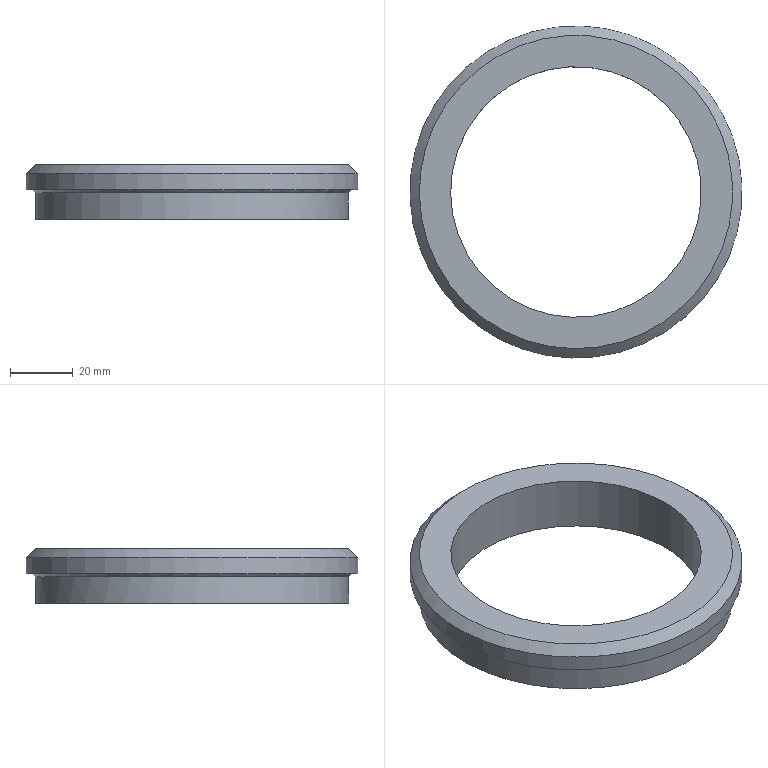Component | NX | CA6140-ZHUZHOU-ZHOUTAO2 | 1 solid | 8 faces | box 106 x 106 x 17.5 mm | volume 55934 mm3 | plane 3 | cylinder 3 | cone 2 | commonest cylinder face diameters 100 x1 80 x1 106 x1
STEP:
#1=CARTESIAN_POINT('',(0.,0.,0.));
#2=DIRECTION('',(0.,0.,1.));
#3=DIRECTION('',(1.,0.,0.));
#4=AXIS2_PLACEMENT_3D('',#1,#2,#3);
#5=CARTESIAN_POINT('',(-29.389,-40.451,-315.951));
#6=VERTEX_POINT('',#5);
#7=CARTESIAN_POINT('',(0.,-0.,-315.951));
#8=DIRECTION('',(0.,0.,1.));
#9=DIRECTION('',(-0.5878,-0.809,0.));
#10=AXIS2_PLACEMENT_3D('',#7,#8,#9);
#11=CIRCLE('',#10,50.);
#12=CARTESIAN_POINT('',(0.,-0.,-315.951));
#13=DIRECTION('',(0.,0.,1.));
#14=DIRECTION('',(-0.5878,-0.809,0.));
#15=AXIS2_PLACEMENT_3D('',#12,#13,#14);
#16=PLANE('',#15);
#17=CARTESIAN_POINT('',(0.,0.));
#18=DIRECTION('',(1.,0.));
#19=AXIS2_PLACEMENT_2D('',#17,#18);
#20=CIRCLE('',#19,50.);
#21=(GEOMETRIC_REPRESENTATION_CONTEXT(2)PARAMETRIC_REPRESENTATION_CONTEXT()REPRESENTATION_CONTEXT('',''));
#22=DEFINITIONAL_REPRESENTATION('',(#20),#21);
#23=PCURVE('',#16,#22);
#24=CARTESIAN_POINT('',(0.,-0.,-318.951));
#25=DIRECTION('',(0.,0.,-1.));
#26=DIRECTION('',(0.5878,0.809,0.));
#27=AXIS2_PLACEMENT_3D('',#24,#25,#26);
#28=CONICAL_SURFACE('',#27,53.,0.7854);
#29=CARTESIAN_POINT('',(9.425,-3.));
#30=DIRECTION('',(-1.,0.));
#31=VECTOR('',#30,1.);
#32=LINE('',#29,#31);
#33=(GEOMETRIC_REPRESENTATION_CONTEXT(2)PARAMETRIC_REPRESENTATION_CONTEXT()REPRESENTATION_CONTEXT('',''));
#34=DEFINITIONAL_REPRESENTATION('',(#32),#33);
#35=PCURVE('',#28,#34);
#36=SURFACE_CURVE('',#11,(#23,#35),.PCURVE_S1.);
#37=EDGE_CURVE('',#6,#6,#36,.T.);
#38=ORIENTED_EDGE('',*,*,#37,.T.);
#39=EDGE_LOOP('',(#38));
#40=FACE_BOUND('',#39,.T.);
#41=CARTESIAN_POINT('',(23.511,32.361,-315.951));
#42=VERTEX_POINT('',#41);
#43=CARTESIAN_POINT('',(0.,-0.,-315.951));
#44=DIRECTION('',(0.,0.,-1.));
#45=DIRECTION('',(0.5878,0.809,0.));
#46=AXIS2_PLACEMENT_3D('',#43,#44,#45);
#47=CIRCLE('',#46,40.);
#48=CARTESIAN_POINT('',(-40.,0.));
#49=CARTESIAN_POINT('',(-40.,69.282));
#50=CARTESIAN_POINT('',(20.,34.641));
#51=CARTESIAN_POINT('',(80.,0.));
#52=CARTESIAN_POINT('',(20.,-34.641));
#53=CARTESIAN_POINT('',(-40.,-69.282));
#54=CARTESIAN_POINT('',(-40.,0.));
#55=(BOUNDED_CURVE()B_SPLINE_CURVE(2,(#48,#49,#50,#51,#52,#53,#54),.UNSPECIFIED.,.T.,.F.)B_SPLINE_CURVE_WITH_KNOTS((1,2,2,2,2,1),(-2.094,0.,2.094,4.189,6.283,8.378),.UNSPECIFIED.)CURVE()GEOMETRIC_REPRESENTATION_ITEM()RATIONAL_B_SPLINE_CURVE((1.,0.5,1.,0.5,1.,0.5,1.))REPRESENTATION_ITEM(''));
#56=(GEOMETRIC_REPRESENTATION_CONTEXT(2)PARAMETRIC_REPRESENTATION_CONTEXT()REPRESENTATION_CONTEXT('',''));
#57=DEFINITIONAL_REPRESENTATION('',(#55),#56);
#58=PCURVE('',#16,#57);
#59=CARTESIAN_POINT('',(0.,-0.,-315.951));
#60=DIRECTION('',(0.,0.,-1.));
#61=DIRECTION('',(0.5878,0.809,0.));
#62=AXIS2_PLACEMENT_3D('',#59,#60,#61);
#63=CYLINDRICAL_SURFACE('',#62,40.);
#64=CARTESIAN_POINT('',(0.,0.));
#65=DIRECTION('',(1.,0.));
#66=VECTOR('',#65,1.);
#67=LINE('',#64,#66);
#68=(GEOMETRIC_REPRESENTATION_CONTEXT(2)PARAMETRIC_REPRESENTATION_CONTEXT()REPRESENTATION_CONTEXT('',''));
#69=DEFINITIONAL_REPRESENTATION('',(#67),#68);
#70=PCURVE('',#63,#69);
#71=SURFACE_CURVE('',#47,(#58,#70),.PCURVE_S1.);
#72=EDGE_CURVE('',#42,#42,#71,.T.);
#73=ORIENTED_EDGE('',*,*,#72,.T.);
#74=EDGE_LOOP('',(#73));
#75=FACE_BOUND('',#74,.T.);
#76=ADVANCED_FACE('',(#40,#75),#16,.T.);
#77=CARTESIAN_POINT('',(23.511,32.361,-333.451));
#78=VERTEX_POINT('',#77);
#79=CARTESIAN_POINT('',(0.,-0.,-333.451));
#80=DIRECTION('',(0.,0.,-1.));
#81=DIRECTION('',(0.5878,0.809,0.));
#82=AXIS2_PLACEMENT_3D('',#79,#80,#81);
#83=CIRCLE('',#82,40.);
#84=CARTESIAN_POINT('',(0.,-0.,-333.451));
#85=DIRECTION('',(0.,0.,-1.));
#86=DIRECTION('',(0.5878,0.809,0.));
#87=AXIS2_PLACEMENT_3D('',#84,#85,#86);
#88=PLANE('',#87);
#89=CARTESIAN_POINT('',(0.,0.));
#90=DIRECTION('',(1.,0.));
#91=AXIS2_PLACEMENT_2D('',#89,#90);
#92=CIRCLE('',#91,40.);
#93=(GEOMETRIC_REPRESENTATION_CONTEXT(2)PARAMETRIC_REPRESENTATION_CONTEXT()REPRESENTATION_CONTEXT('',''));
#94=DEFINITIONAL_REPRESENTATION('',(#92),#93);
#95=PCURVE('',#88,#94);
#96=CARTESIAN_POINT('',(0.,17.5));
#97=DIRECTION('',(1.,0.));
#98=VECTOR('',#97,1.);
#99=LINE('',#96,#98);
#100=(GEOMETRIC_REPRESENTATION_CONTEXT(2)PARAMETRIC_REPRESENTATION_CONTEXT()REPRESENTATION_CONTEXT('',''));
#101=DEFINITIONAL_REPRESENTATION('',(#99),#100);
#102=PCURVE('',#63,#101);
#103=SURFACE_CURVE('',#83,(#95,#102),.PCURVE_S1.);
#104=EDGE_CURVE('',#78,#78,#103,.T.);
#105=ORIENTED_EDGE('',*,*,#104,.F.);
#106=EDGE_LOOP('',(#105));
#107=FACE_BOUND('',#106,.T.);
#108=CARTESIAN_POINT('',(-29.389,-40.451,-333.451));
#109=VERTEX_POINT('',#108);
#110=CARTESIAN_POINT('',(0.,-0.,-333.451));
#111=DIRECTION('',(0.,0.,1.));
#112=DIRECTION('',(-0.5878,-0.809,0.));
#113=AXIS2_PLACEMENT_3D('',#110,#111,#112);
#114=CIRCLE('',#113,50.);
#115=CARTESIAN_POINT('',(-50.,0.));
#116=CARTESIAN_POINT('',(-50.,86.603));
#117=CARTESIAN_POINT('',(25.,43.301));
#118=CARTESIAN_POINT('',(100.,0.));
#119=CARTESIAN_POINT('',(25.,-43.301));
#120=CARTESIAN_POINT('',(-50.,-86.603));
#121=CARTESIAN_POINT('',(-50.,0.));
#122=(BOUNDED_CURVE()B_SPLINE_CURVE(2,(#115,#116,#117,#118,#119,#120,#121),.UNSPECIFIED.,.T.,.F.)B_SPLINE_CURVE_WITH_KNOTS((1,2,2,2,2,1),(-2.094,0.,2.094,4.189,6.283,8.378),.UNSPECIFIED.)CURVE()GEOMETRIC_REPRESENTATION_ITEM()RATIONAL_B_SPLINE_CURVE((1.,0.5,1.,0.5,1.,0.5,1.))REPRESENTATION_ITEM(''));
#123=(GEOMETRIC_REPRESENTATION_CONTEXT(2)PARAMETRIC_REPRESENTATION_CONTEXT()REPRESENTATION_CONTEXT('',''));
#124=DEFINITIONAL_REPRESENTATION('',(#122),#123);
#125=PCURVE('',#88,#124);
#126=CARTESIAN_POINT('',(0.,-0.,-333.451));
#127=DIRECTION('',(0.,0.,1.));
#128=DIRECTION('',(-0.5878,-0.809,0.));
#129=AXIS2_PLACEMENT_3D('',#126,#127,#128);
#130=CYLINDRICAL_SURFACE('',#129,50.);
#131=CARTESIAN_POINT('',(0.,0.));
#132=DIRECTION('',(1.,0.));
#133=VECTOR('',#132,1.);
#134=LINE('',#131,#133);
#135=(GEOMETRIC_REPRESENTATION_CONTEXT(2)PARAMETRIC_REPRESENTATION_CONTEXT()REPRESENTATION_CONTEXT('',''));
#136=DEFINITIONAL_REPRESENTATION('',(#134),#135);
#137=PCURVE('',#130,#136);
#138=SURFACE_CURVE('',#114,(#125,#137),.PCURVE_S1.);
#139=EDGE_CURVE('',#109,#109,#138,.T.);
#140=ORIENTED_EDGE('',*,*,#139,.F.);
#141=EDGE_LOOP('',(#140));
#142=FACE_BOUND('',#141,.T.);
#143=ADVANCED_FACE('',(#107,#142),#88,.T.);
#144=CARTESIAN_POINT('',(29.389,40.451,-324.951));
#145=VERTEX_POINT('',#144);
#146=CARTESIAN_POINT('',(-29.389,-40.451,-324.951));
#147=VERTEX_POINT('',#146);
#148=CARTESIAN_POINT('',(0.,-0.,-324.951));
#149=DIRECTION('',(0.,0.,-1.));
#150=DIRECTION('',(0.5878,0.809,0.));
#151=AXIS2_PLACEMENT_3D('',#148,#149,#150);
#152=CIRCLE('',#151,50.);
#153=CARTESIAN_POINT('',(3.142,8.5));
#154=DIRECTION('',(-1.,0.));
#155=VECTOR('',#154,1.);
#156=LINE('',#153,#155);
#157=(GEOMETRIC_REPRESENTATION_CONTEXT(2)PARAMETRIC_REPRESENTATION_CONTEXT()REPRESENTATION_CONTEXT('',''));
#158=DEFINITIONAL_REPRESENTATION('',(#156),#157);
#159=PCURVE('',#130,#158);
#160=CARTESIAN_POINT('',(0.,-0.,-323.951));
#161=DIRECTION('',(0.,0.,1.));
#162=DIRECTION('',(-0.5878,-0.809,0.));
#163=AXIS2_PLACEMENT_3D('',#160,#161,#162);
#164=CONICAL_SURFACE('',#163,51.,0.7854);
#165=CARTESIAN_POINT('',(3.142,-1.));
#166=DIRECTION('',(-1.,0.));
#167=VECTOR('',#166,1.);
#168=LINE('',#165,#167);
#169=(GEOMETRIC_REPRESENTATION_CONTEXT(2)PARAMETRIC_REPRESENTATION_CONTEXT()REPRESENTATION_CONTEXT('',''));
#170=DEFINITIONAL_REPRESENTATION('',(#168),#169);
#171=PCURVE('',#164,#170);
#172=SURFACE_CURVE('',#152,(#159,#171),.PCURVE_S1.);
#173=EDGE_CURVE('',#145,#147,#172,.T.);
#174=ORIENTED_EDGE('',*,*,#173,.T.);
#175=CARTESIAN_POINT('',(-29.389,-40.451,-333.451));
#176=CARTESIAN_POINT('',(-29.389,-40.451,-324.951));
#177=B_SPLINE_CURVE_WITH_KNOTS('',1,(#175,#176),.UNSPECIFIED.,.F.,.F.,(2,2),(0.,8.5),.PIECEWISE_BEZIER_KNOTS.);
#178=CARTESIAN_POINT('',(0.,0.));
#179=DIRECTION('',(0.,1.));
#180=VECTOR('',#179,1.);
#181=LINE('',#178,#180);
#182=(GEOMETRIC_REPRESENTATION_CONTEXT(2)PARAMETRIC_REPRESENTATION_CONTEXT()REPRESENTATION_CONTEXT('',''));
#183=DEFINITIONAL_REPRESENTATION('',(#181),#182);
#184=PCURVE('',#130,#183);
#185=CARTESIAN_POINT('',(6.283,0.));
#186=DIRECTION('',(0.,1.));
#187=VECTOR('',#186,1.);
#188=LINE('',#185,#187);
#189=(GEOMETRIC_REPRESENTATION_CONTEXT(2)PARAMETRIC_REPRESENTATION_CONTEXT()REPRESENTATION_CONTEXT('',''));
#190=DEFINITIONAL_REPRESENTATION('',(#188),#189);
#191=PCURVE('',#130,#190);
#192=SEAM_CURVE('',#177,(#184,#191),.PCURVE_S1.);
#193=EDGE_CURVE('',#109,#147,#192,.T.);
#194=ORIENTED_EDGE('',*,*,#193,.F.);
#195=ORIENTED_EDGE('',*,*,#139,.T.);
#196=ORIENTED_EDGE('',*,*,#193,.T.);
#197=CARTESIAN_POINT('',(0.,-0.,-324.951));
#198=DIRECTION('',(0.,0.,-1.));
#199=DIRECTION('',(0.5878,0.809,0.));
#200=AXIS2_PLACEMENT_3D('',#197,#198,#199);
#201=CIRCLE('',#200,50.);
#202=CARTESIAN_POINT('',(9.425,8.5));
#203=DIRECTION('',(-1.,0.));
#204=VECTOR('',#203,1.);
#205=LINE('',#202,#204);
#206=(GEOMETRIC_REPRESENTATION_CONTEXT(2)PARAMETRIC_REPRESENTATION_CONTEXT()REPRESENTATION_CONTEXT('',''));
#207=DEFINITIONAL_REPRESENTATION('',(#205),#206);
#208=PCURVE('',#130,#207);
#209=CARTESIAN_POINT('',(9.425,-1.));
#210=DIRECTION('',(-1.,0.));
#211=VECTOR('',#210,1.);
#212=LINE('',#209,#211);
#213=(GEOMETRIC_REPRESENTATION_CONTEXT(2)PARAMETRIC_REPRESENTATION_CONTEXT()REPRESENTATION_CONTEXT('',''));
#214=DEFINITIONAL_REPRESENTATION('',(#212),#213);
#215=PCURVE('',#164,#214);
#216=SURFACE_CURVE('',#201,(#208,#215),.PCURVE_S1.);
#217=EDGE_CURVE('',#147,#145,#216,.T.);
#218=ORIENTED_EDGE('',*,*,#217,.T.);
#219=EDGE_LOOP('',(#174,#194,#195,#196,#218));
#220=FACE_BOUND('',#219,.T.);
#221=ADVANCED_FACE('',(#220),#130,.T.);
#222=ORIENTED_EDGE('',*,*,#104,.F.);
#223=CARTESIAN_POINT('',(23.511,32.361,-315.951));
#224=CARTESIAN_POINT('',(23.511,32.361,-333.451));
#225=B_SPLINE_CURVE_WITH_KNOTS('',1,(#223,#224),.UNSPECIFIED.,.F.,.F.,(2,2),(0.,17.5),.PIECEWISE_BEZIER_KNOTS.);
#226=CARTESIAN_POINT('',(0.,0.));
#227=DIRECTION('',(0.,1.));
#228=VECTOR('',#227,1.);
#229=LINE('',#226,#228);
#230=(GEOMETRIC_REPRESENTATION_CONTEXT(2)PARAMETRIC_REPRESENTATION_CONTEXT()REPRESENTATION_CONTEXT('',''));
#231=DEFINITIONAL_REPRESENTATION('',(#229),#230);
#232=PCURVE('',#63,#231);
#233=CARTESIAN_POINT('',(6.283,0.));
#234=DIRECTION('',(0.,1.));
#235=VECTOR('',#234,1.);
#236=LINE('',#233,#235);
#237=(GEOMETRIC_REPRESENTATION_CONTEXT(2)PARAMETRIC_REPRESENTATION_CONTEXT()REPRESENTATION_CONTEXT('',''));
#238=DEFINITIONAL_REPRESENTATION('',(#236),#237);
#239=PCURVE('',#63,#238);
#240=SEAM_CURVE('',#225,(#232,#239),.PCURVE_S1.);
#241=EDGE_CURVE('',#42,#78,#240,.T.);
#242=ORIENTED_EDGE('',*,*,#241,.F.);
#243=ORIENTED_EDGE('',*,*,#72,.T.);
#244=ORIENTED_EDGE('',*,*,#241,.T.);
#245=EDGE_LOOP('',(#222,#242,#243,#244));
#246=FACE_BOUND('',#245,.F.);
#247=ADVANCED_FACE('',(#246),#63,.F.);
#248=CARTESIAN_POINT('',(-29.977,-41.26,-323.951));
#249=VERTEX_POINT('',#248);
#250=CARTESIAN_POINT('',(0.,-0.,-323.951));
#251=DIRECTION('',(0.,0.,1.));
#252=DIRECTION('',(-0.5878,-0.809,0.));
#253=AXIS2_PLACEMENT_3D('',#250,#251,#252);
#254=CIRCLE('',#253,51.);
#255=CARTESIAN_POINT('',(0.,-0.,-323.951));
#256=DIRECTION('',(0.,0.,1.));
#257=DIRECTION('',(-0.5878,-0.809,0.));
#258=AXIS2_PLACEMENT_3D('',#255,#256,#257);
#259=PLANE('',#258);
#260=CARTESIAN_POINT('',(0.,0.));
#261=DIRECTION('',(1.,0.));
#262=AXIS2_PLACEMENT_2D('',#260,#261);
#263=CIRCLE('',#262,51.);
#264=(GEOMETRIC_REPRESENTATION_CONTEXT(2)PARAMETRIC_REPRESENTATION_CONTEXT()REPRESENTATION_CONTEXT('',''));
#265=DEFINITIONAL_REPRESENTATION('',(#263),#264);
#266=PCURVE('',#259,#265);
#267=CARTESIAN_POINT('',(0.,0.));
#268=DIRECTION('',(1.,0.));
#269=VECTOR('',#268,1.);
#270=LINE('',#267,#269);
#271=(GEOMETRIC_REPRESENTATION_CONTEXT(2)PARAMETRIC_REPRESENTATION_CONTEXT()REPRESENTATION_CONTEXT('',''));
#272=DEFINITIONAL_REPRESENTATION('',(#270),#271);
#273=PCURVE('',#164,#272);
#274=SURFACE_CURVE('',#254,(#266,#273),.PCURVE_S1.);
#275=EDGE_CURVE('',#249,#249,#274,.T.);
#276=ORIENTED_EDGE('',*,*,#275,.T.);
#277=EDGE_LOOP('',(#276));
#278=FACE_BOUND('',#277,.T.);
#279=CARTESIAN_POINT('',(31.153,42.878,-323.951));
#280=VERTEX_POINT('',#279);
#281=CARTESIAN_POINT('',(0.,-0.,-323.951));
#282=DIRECTION('',(0.,0.,-1.));
#283=DIRECTION('',(0.5878,0.809,0.));
#284=AXIS2_PLACEMENT_3D('',#281,#282,#283);
#285=CIRCLE('',#284,53.);
#286=CARTESIAN_POINT('',(-53.,0.));
#287=CARTESIAN_POINT('',(-53.,91.799));
#288=CARTESIAN_POINT('',(26.5,45.899));
#289=CARTESIAN_POINT('',(106.,0.));
#290=CARTESIAN_POINT('',(26.5,-45.899));
#291=CARTESIAN_POINT('',(-53.,-91.799));
#292=CARTESIAN_POINT('',(-53.,0.));
#293=(BOUNDED_CURVE()B_SPLINE_CURVE(2,(#286,#287,#288,#289,#290,#291,#292),.UNSPECIFIED.,.T.,.F.)B_SPLINE_CURVE_WITH_KNOTS((1,2,2,2,2,1),(-2.094,0.,2.094,4.189,6.283,8.378),.UNSPECIFIED.)CURVE()GEOMETRIC_REPRESENTATION_ITEM()RATIONAL_B_SPLINE_CURVE((1.,0.5,1.,0.5,1.,0.5,1.))REPRESENTATION_ITEM(''));
#294=(GEOMETRIC_REPRESENTATION_CONTEXT(2)PARAMETRIC_REPRESENTATION_CONTEXT()REPRESENTATION_CONTEXT('',''));
#295=DEFINITIONAL_REPRESENTATION('',(#293),#294);
#296=PCURVE('',#259,#295);
#297=CARTESIAN_POINT('',(0.,-0.,-315.951));
#298=DIRECTION('',(0.,0.,-1.));
#299=DIRECTION('',(0.5878,0.809,0.));
#300=AXIS2_PLACEMENT_3D('',#297,#298,#299);
#301=CYLINDRICAL_SURFACE('',#300,53.);
#302=CARTESIAN_POINT('',(0.,8.));
#303=DIRECTION('',(1.,0.));
#304=VECTOR('',#303,1.);
#305=LINE('',#302,#304);
#306=(GEOMETRIC_REPRESENTATION_CONTEXT(2)PARAMETRIC_REPRESENTATION_CONTEXT()REPRESENTATION_CONTEXT('',''));
#307=DEFINITIONAL_REPRESENTATION('',(#305),#306);
#308=PCURVE('',#301,#307);
#309=SURFACE_CURVE('',#285,(#296,#308),.PCURVE_S1.);
#310=EDGE_CURVE('',#280,#280,#309,.T.);
#311=ORIENTED_EDGE('',*,*,#310,.T.);
#312=EDGE_LOOP('',(#311));
#313=FACE_BOUND('',#312,.T.);
#314=ADVANCED_FACE('',(#278,#313),#259,.F.);
#315=CARTESIAN_POINT('',(-31.153,-42.878,-318.951));
#316=VERTEX_POINT('',#315);
#317=CARTESIAN_POINT('',(31.153,42.878,-318.951));
#318=VERTEX_POINT('',#317);
#319=CARTESIAN_POINT('',(0.,-0.,-318.951));
#320=DIRECTION('',(0.,0.,-1.));
#321=DIRECTION('',(-0.5878,-0.809,0.));
#322=AXIS2_PLACEMENT_3D('',#319,#320,#321);
#323=CIRCLE('',#322,53.);
#324=CARTESIAN_POINT('',(3.142,3.));
#325=DIRECTION('',(1.,0.));
#326=VECTOR('',#325,1.);
#327=LINE('',#324,#326);
#328=(GEOMETRIC_REPRESENTATION_CONTEXT(2)PARAMETRIC_REPRESENTATION_CONTEXT()REPRESENTATION_CONTEXT('',''));
#329=DEFINITIONAL_REPRESENTATION('',(#327),#328);
#330=PCURVE('',#301,#329);
#331=CARTESIAN_POINT('',(3.142,0.));
#332=DIRECTION('',(1.,0.));
#333=VECTOR('',#332,1.);
#334=LINE('',#331,#333);
#335=(GEOMETRIC_REPRESENTATION_CONTEXT(2)PARAMETRIC_REPRESENTATION_CONTEXT()REPRESENTATION_CONTEXT('',''));
#336=DEFINITIONAL_REPRESENTATION('',(#334),#335);
#337=PCURVE('',#28,#336);
#338=SURFACE_CURVE('',#323,(#330,#337),.PCURVE_S1.);
#339=EDGE_CURVE('',#316,#318,#338,.T.);
#340=ORIENTED_EDGE('',*,*,#339,.T.);
#341=CARTESIAN_POINT('',(31.153,42.878,-318.951));
#342=CARTESIAN_POINT('',(31.153,42.878,-323.951));
#343=B_SPLINE_CURVE_WITH_KNOTS('',1,(#341,#342),.UNSPECIFIED.,.F.,.F.,(2,2),(3.,8.),.PIECEWISE_BEZIER_KNOTS.);
#344=CARTESIAN_POINT('',(6.283,0.));
#345=DIRECTION('',(0.,1.));
#346=VECTOR('',#345,1.);
#347=LINE('',#344,#346);
#348=(GEOMETRIC_REPRESENTATION_CONTEXT(2)PARAMETRIC_REPRESENTATION_CONTEXT()REPRESENTATION_CONTEXT('',''));
#349=DEFINITIONAL_REPRESENTATION('',(#347),#348);
#350=PCURVE('',#301,#349);
#351=CARTESIAN_POINT('',(0.,0.));
#352=DIRECTION('',(0.,1.));
#353=VECTOR('',#352,1.);
#354=LINE('',#351,#353);
#355=(GEOMETRIC_REPRESENTATION_CONTEXT(2)PARAMETRIC_REPRESENTATION_CONTEXT()REPRESENTATION_CONTEXT('',''));
#356=DEFINITIONAL_REPRESENTATION('',(#354),#355);
#357=PCURVE('',#301,#356);
#358=SEAM_CURVE('',#343,(#350,#357),.PCURVE_S1.);
#359=EDGE_CURVE('',#318,#280,#358,.T.);
#360=ORIENTED_EDGE('',*,*,#359,.T.);
#361=ORIENTED_EDGE('',*,*,#310,.F.);
#362=ORIENTED_EDGE('',*,*,#359,.F.);
#363=CARTESIAN_POINT('',(0.,-0.,-318.951));
#364=DIRECTION('',(0.,0.,-1.));
#365=DIRECTION('',(-0.5878,-0.809,0.));
#366=AXIS2_PLACEMENT_3D('',#363,#364,#365);
#367=CIRCLE('',#366,53.);
#368=CARTESIAN_POINT('',(-3.142,3.));
#369=DIRECTION('',(1.,0.));
#370=VECTOR('',#369,1.);
#371=LINE('',#368,#370);
#372=(GEOMETRIC_REPRESENTATION_CONTEXT(2)PARAMETRIC_REPRESENTATION_CONTEXT()REPRESENTATION_CONTEXT('',''));
#373=DEFINITIONAL_REPRESENTATION('',(#371),#372);
#374=PCURVE('',#301,#373);
#375=CARTESIAN_POINT('',(3.142,0.));
#376=DIRECTION('',(1.,-0.));
#377=VECTOR('',#376,1.);
#378=LINE('',#375,#377);
#379=(GEOMETRIC_REPRESENTATION_CONTEXT(2)PARAMETRIC_REPRESENTATION_CONTEXT()REPRESENTATION_CONTEXT('',''));
#380=DEFINITIONAL_REPRESENTATION('',(#378),#379);
#381=PCURVE('',#28,#380);
#382=SURFACE_CURVE('',#367,(#374,#381),.PCURVE_S1.);
#383=EDGE_CURVE('',#318,#316,#382,.T.);
#384=ORIENTED_EDGE('',*,*,#383,.T.);
#385=EDGE_LOOP('',(#340,#360,#361,#362,#384));
#386=FACE_BOUND('',#385,.T.);
#387=ADVANCED_FACE('',(#386),#301,.T.);
#388=ORIENTED_EDGE('',*,*,#37,.F.);
#389=CARTESIAN_POINT('',(-29.389,-40.451,-315.951));
#390=CARTESIAN_POINT('',(-31.153,-42.878,-318.951));
#391=B_SPLINE_CURVE_WITH_KNOTS('',1,(#389,#390),.UNSPECIFIED.,.F.,.F.,(2,2),(-4.243,0.),.PIECEWISE_BEZIER_KNOTS.);
#392=CARTESIAN_POINT('',(9.425,0.));
#393=DIRECTION('',(0.,1.));
#394=VECTOR('',#393,1.);
#395=LINE('',#392,#394);
#396=(GEOMETRIC_REPRESENTATION_CONTEXT(2)PARAMETRIC_REPRESENTATION_CONTEXT()REPRESENTATION_CONTEXT('',''));
#397=DEFINITIONAL_REPRESENTATION('',(#395),#396);
#398=PCURVE('',#28,#397);
#399=CARTESIAN_POINT('',(3.142,0.));
#400=DIRECTION('',(0.,1.));
#401=VECTOR('',#400,1.);
#402=LINE('',#399,#401);
#403=(GEOMETRIC_REPRESENTATION_CONTEXT(2)PARAMETRIC_REPRESENTATION_CONTEXT()REPRESENTATION_CONTEXT('',''));
#404=DEFINITIONAL_REPRESENTATION('',(#402),#403);
#405=PCURVE('',#28,#404);
#406=SEAM_CURVE('',#391,(#398,#405),.PCURVE_S1.);
#407=EDGE_CURVE('',#6,#316,#406,.T.);
#408=ORIENTED_EDGE('',*,*,#407,.T.);
#409=ORIENTED_EDGE('',*,*,#383,.F.);
#410=ORIENTED_EDGE('',*,*,#339,.F.);
#411=ORIENTED_EDGE('',*,*,#407,.F.);
#412=EDGE_LOOP('',(#388,#408,#409,#410,#411));
#413=FACE_BOUND('',#412,.T.);
#414=ADVANCED_FACE('',(#413),#28,.T.);
#415=ORIENTED_EDGE('',*,*,#173,.F.);
#416=ORIENTED_EDGE('',*,*,#217,.F.);
#417=CARTESIAN_POINT('',(-29.389,-40.451,-324.951));
#418=CARTESIAN_POINT('',(-29.977,-41.26,-323.951));
#419=B_SPLINE_CURVE_WITH_KNOTS('',1,(#417,#418),.UNSPECIFIED.,.F.,.F.,(2,2),(-1.414,0.),.PIECEWISE_BEZIER_KNOTS.);
#420=CARTESIAN_POINT('',(6.283,0.));
#421=DIRECTION('',(0.,1.));
#422=VECTOR('',#421,1.);
#423=LINE('',#420,#422);
#424=(GEOMETRIC_REPRESENTATION_CONTEXT(2)PARAMETRIC_REPRESENTATION_CONTEXT()REPRESENTATION_CONTEXT('',''));
#425=DEFINITIONAL_REPRESENTATION('',(#423),#424);
#426=PCURVE('',#164,#425);
#427=CARTESIAN_POINT('',(0.,0.));
#428=DIRECTION('',(0.,1.));
#429=VECTOR('',#428,1.);
#430=LINE('',#427,#429);
#431=(GEOMETRIC_REPRESENTATION_CONTEXT(2)PARAMETRIC_REPRESENTATION_CONTEXT()REPRESENTATION_CONTEXT('',''));
#432=DEFINITIONAL_REPRESENTATION('',(#430),#431);
#433=PCURVE('',#164,#432);
#434=SEAM_CURVE('',#419,(#426,#433),.PCURVE_S1.);
#435=EDGE_CURVE('',#147,#249,#434,.T.);
#436=ORIENTED_EDGE('',*,*,#435,.T.);
#437=ORIENTED_EDGE('',*,*,#275,.F.);
#438=ORIENTED_EDGE('',*,*,#435,.F.);
#439=EDGE_LOOP('',(#415,#416,#436,#437,#438));
#440=FACE_BOUND('',#439,.T.);
#441=ADVANCED_FACE('',(#440),#164,.T.);
#442=CLOSED_SHELL('',(#76,#143,#221,#247,#314,#387,#414,#441));
#443=MANIFOLD_SOLID_BREP('',#442);
#444=(LENGTH_UNIT()NAMED_UNIT(*)SI_UNIT(.MILLI.,.METRE.));
#445=UNCERTAINTY_MEASURE_WITH_UNIT(LENGTH_MEASURE(0.00001),#444,'','');
#446=(NAMED_UNIT(*)PLANE_ANGLE_UNIT()SI_UNIT($,.RADIAN.));
#447=(NAMED_UNIT(*)SI_UNIT($,.STERADIAN.)SOLID_ANGLE_UNIT());
#448=(GEOMETRIC_REPRESENTATION_CONTEXT(3)GLOBAL_UNCERTAINTY_ASSIGNED_CONTEXT((#445))GLOBAL_UNIT_ASSIGNED_CONTEXT((#444,#446,#447))REPRESENTATION_CONTEXT('',''));
#449=ADVANCED_BREP_SHAPE_REPRESENTATION('',(#4,#443),#448);